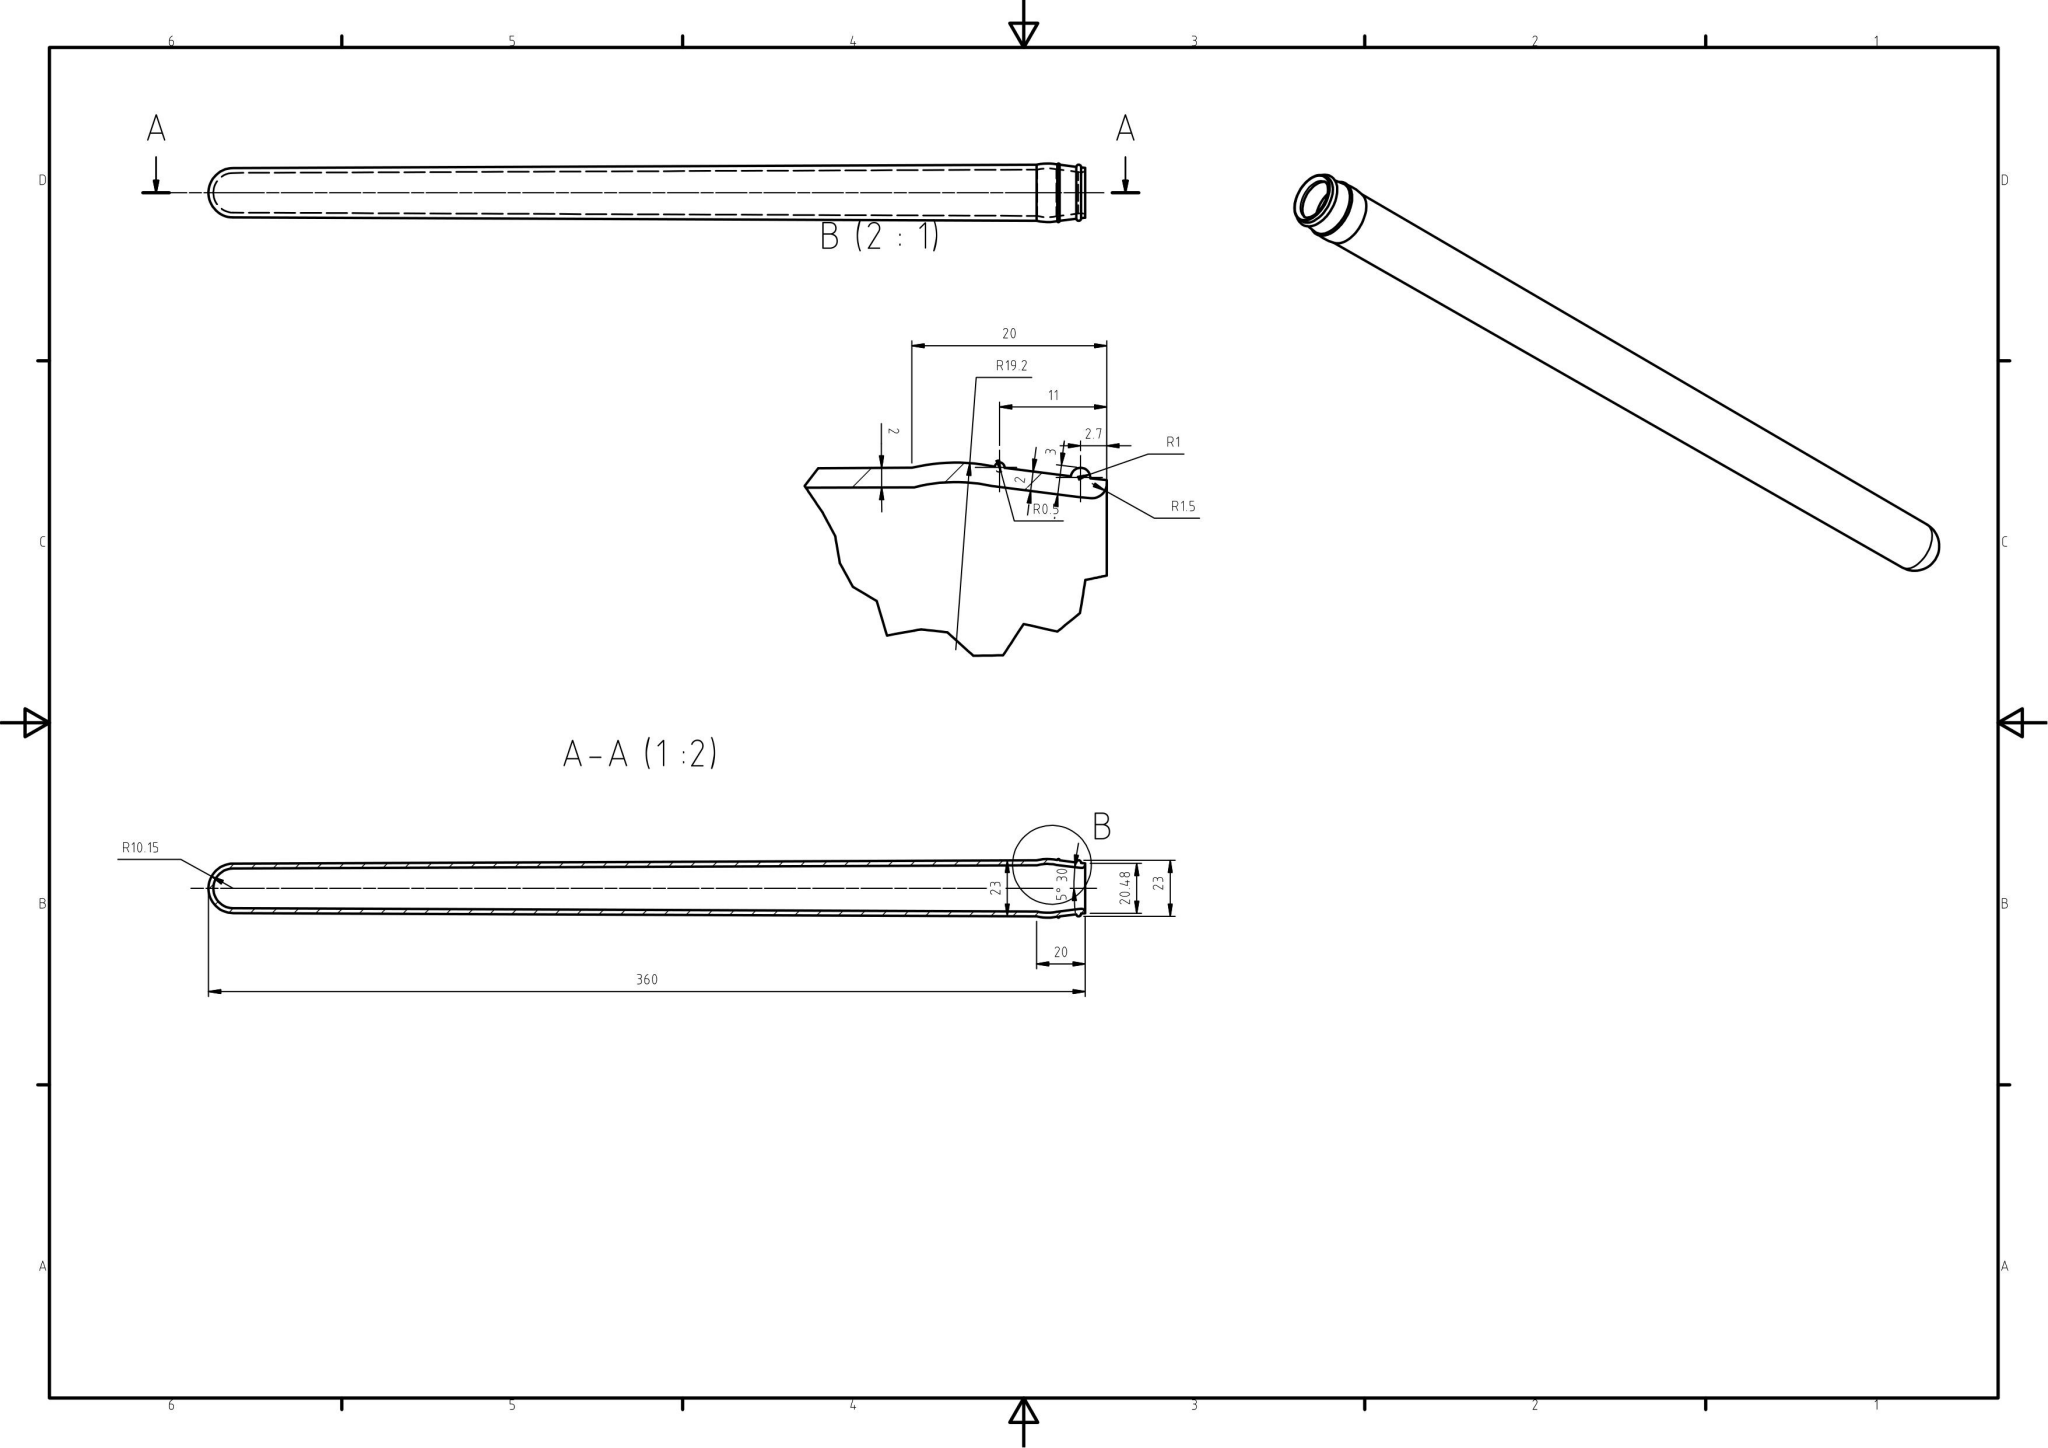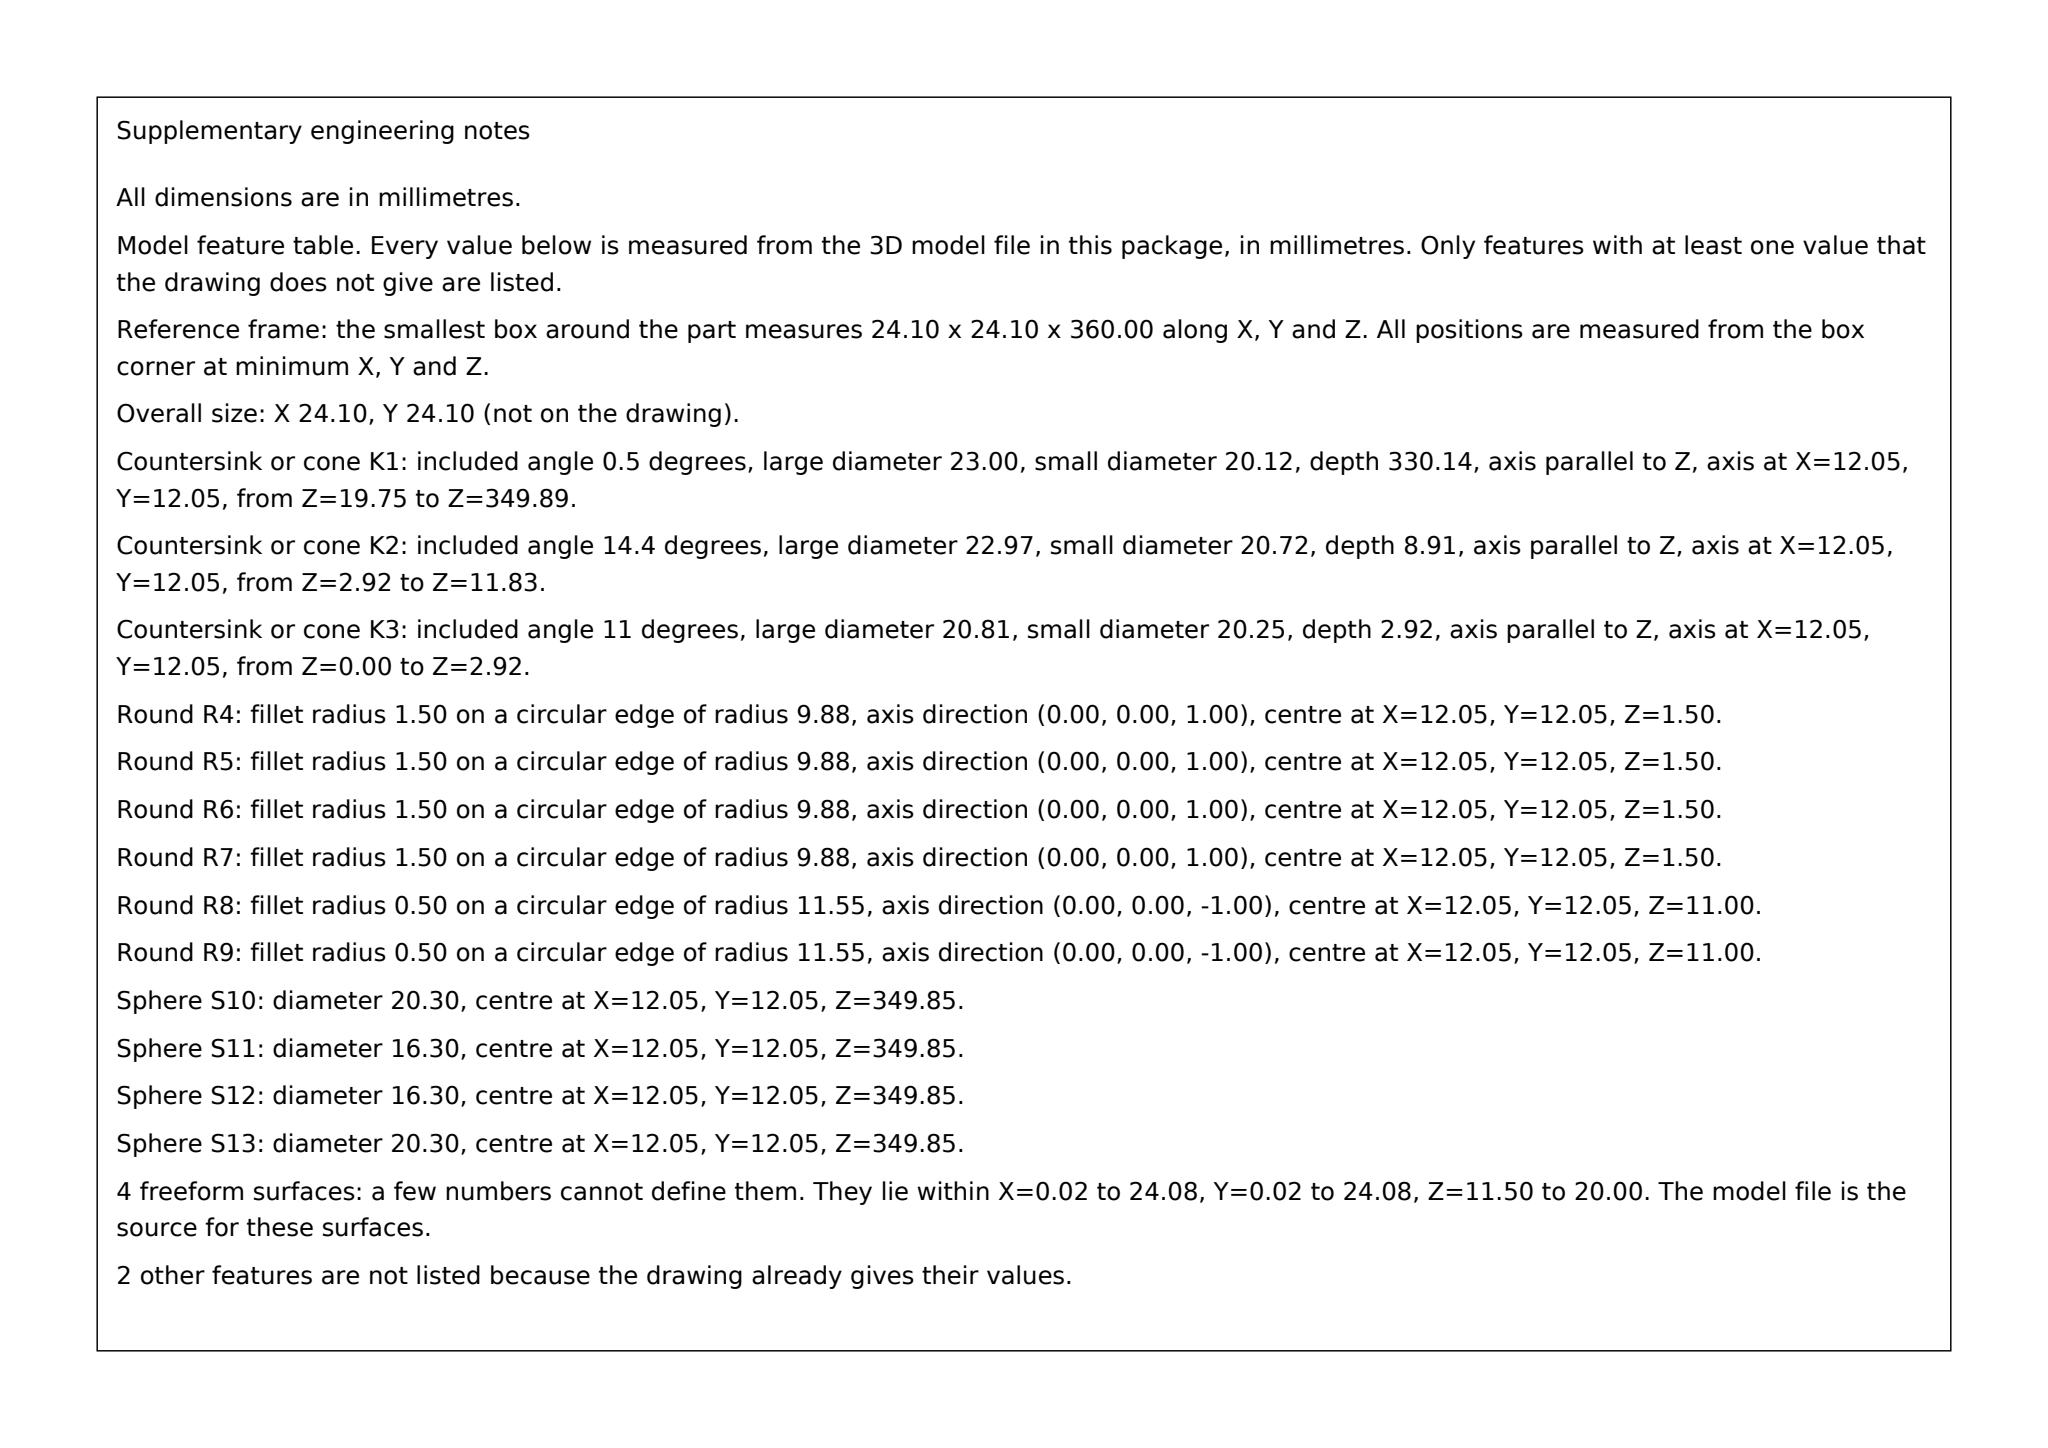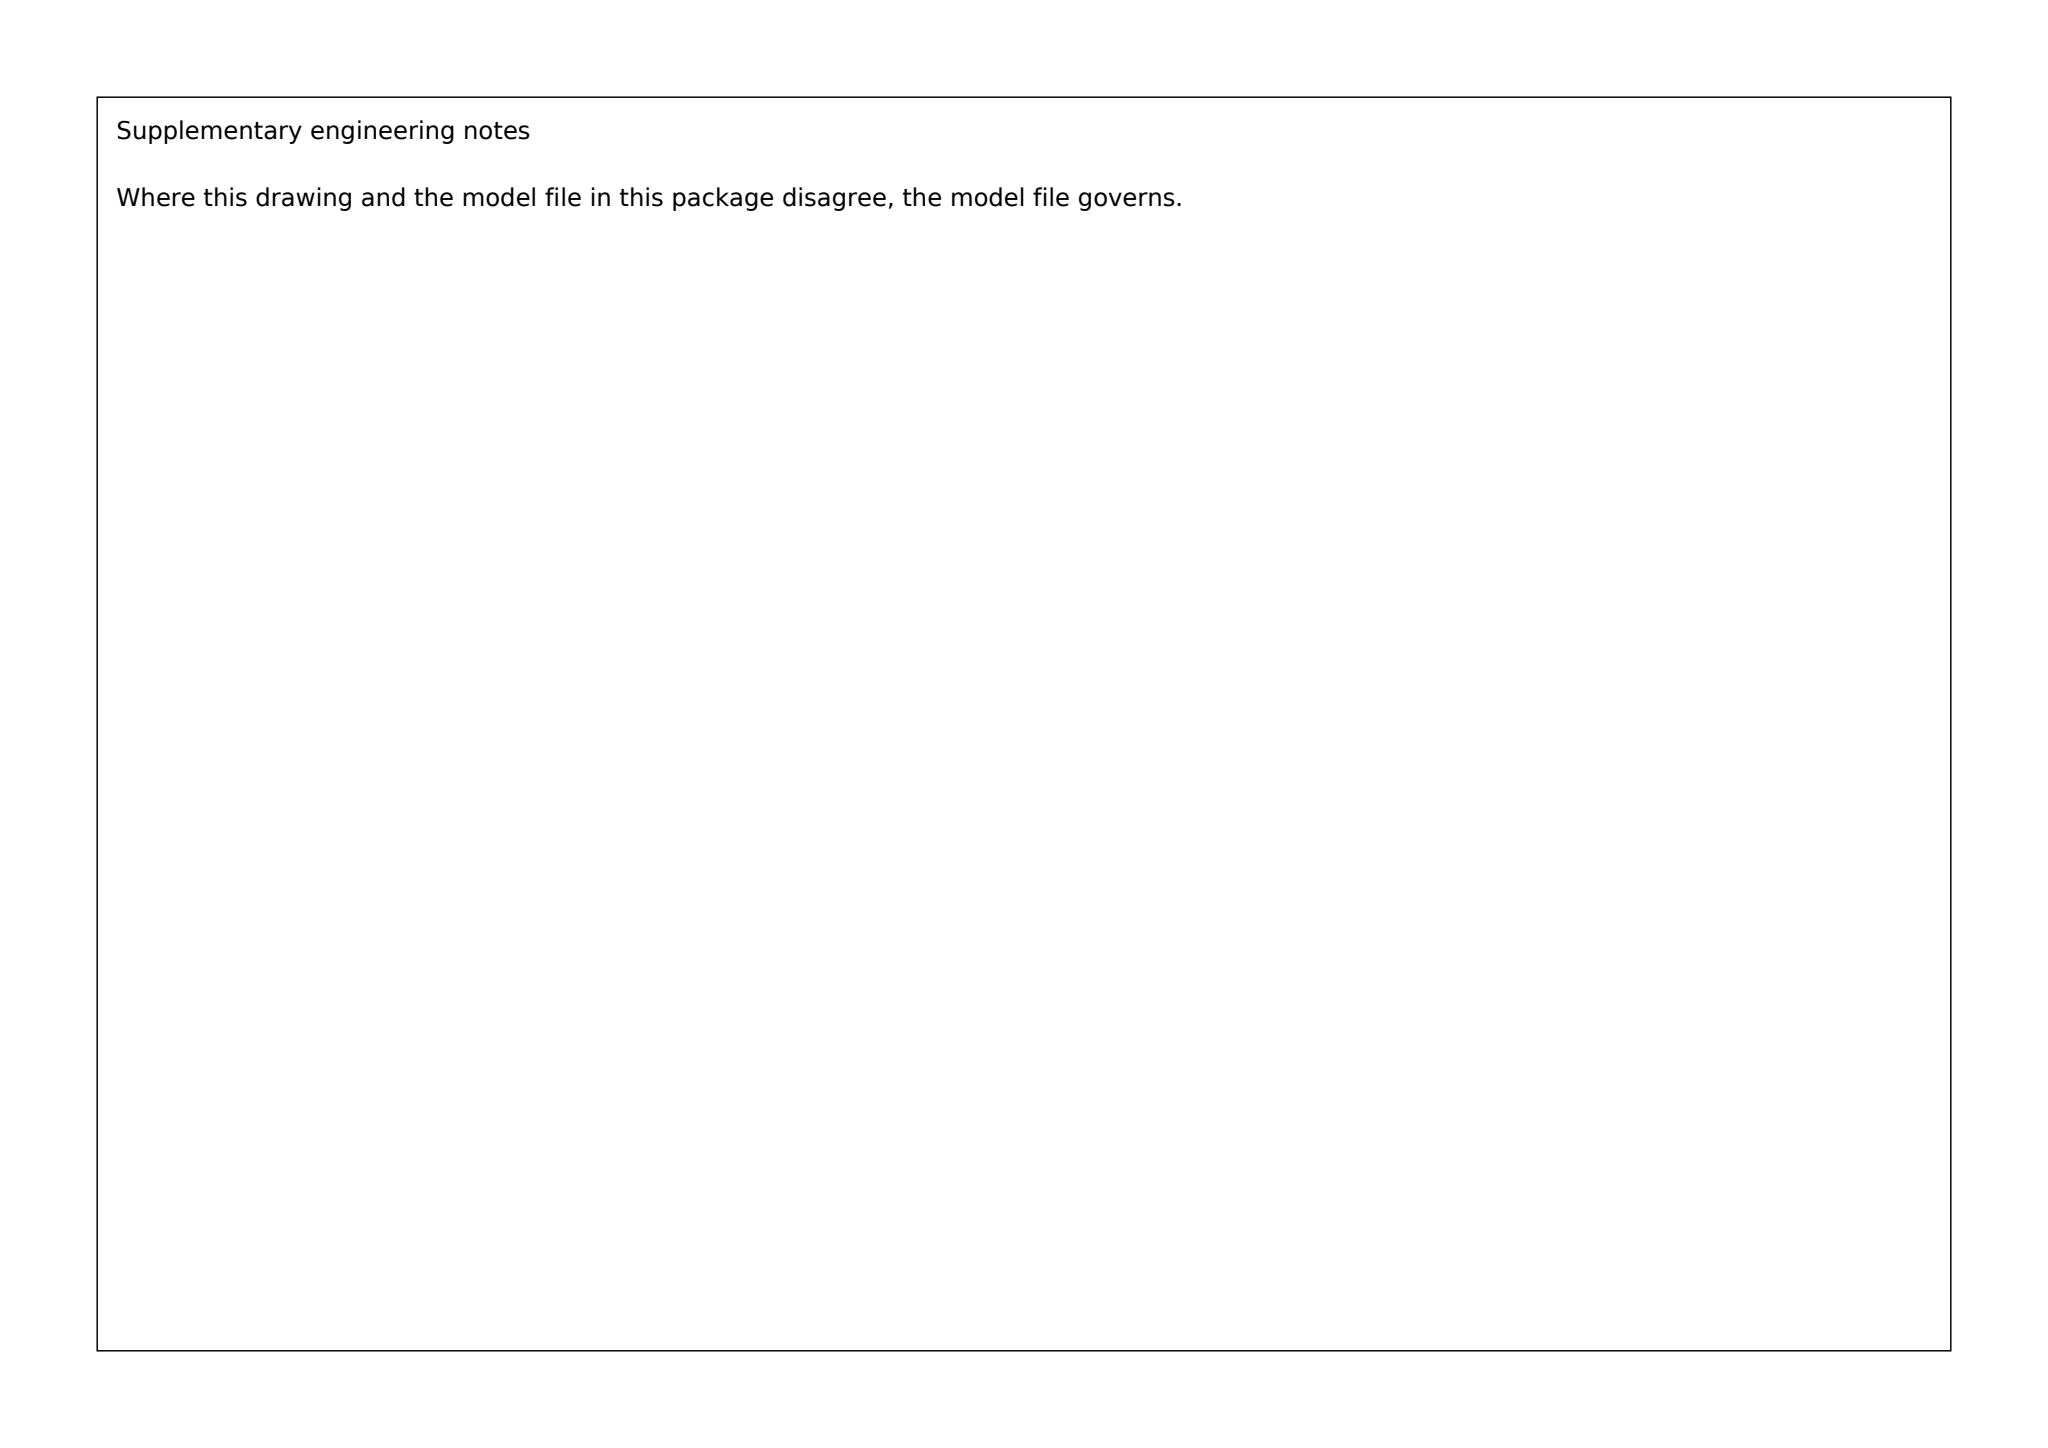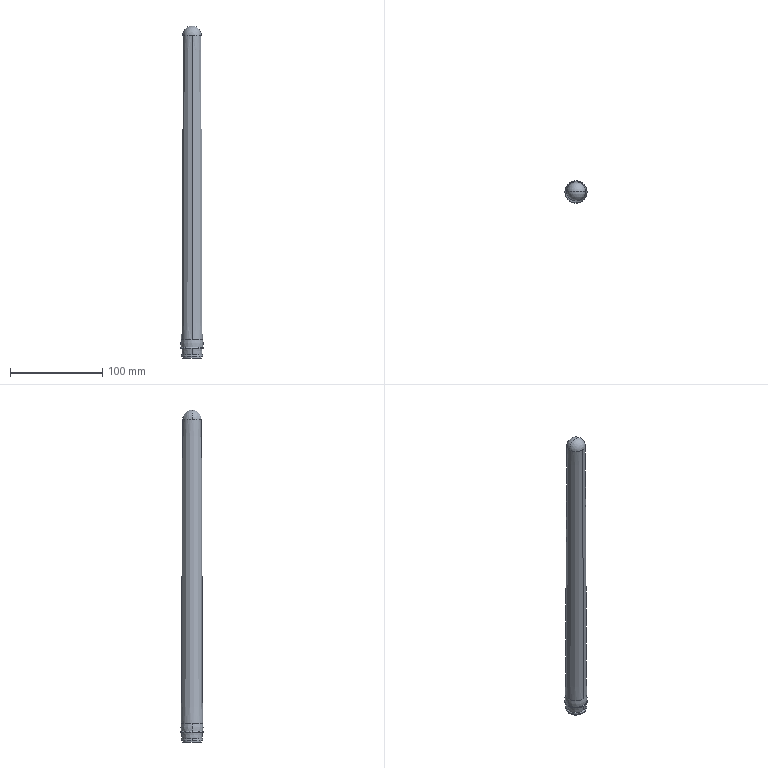Part | SolidWorks | mm | 1 solid | 29 faces | box 24.1 x 24.1 x 360 mm | volume 44494 mm3 | cone 12 | torus 8 | spline 4 | sphere 4 | plane 1